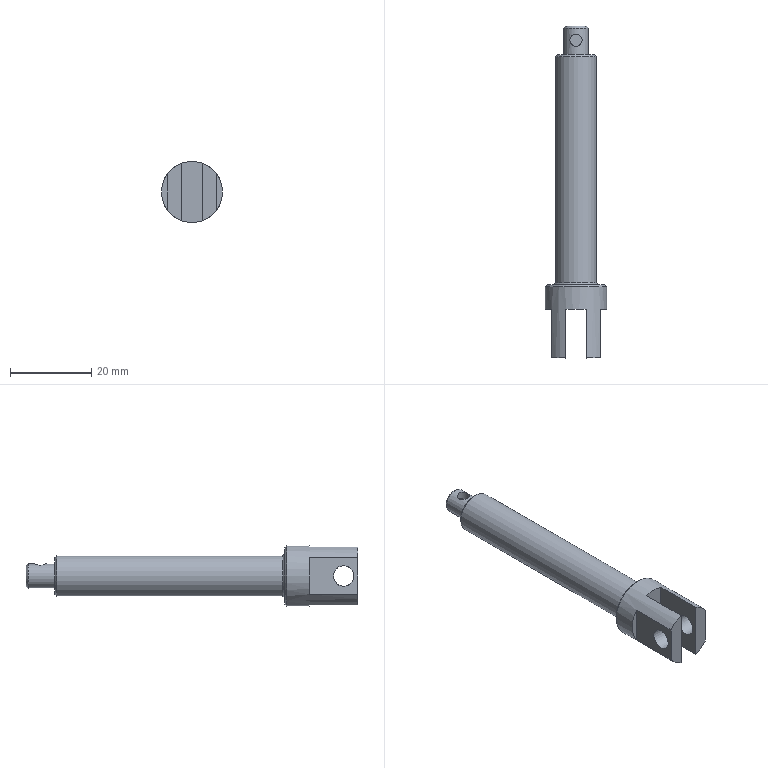Component | NX | PUSH_ROD | 1 solid | 26 faces | volume 6512 mm3 | plane 14 | cylinder 8 | cone 4 | commonest cylinder face diameters 5 x2 2.5 x2 15 x1 10 x1 6 x1 3 x1